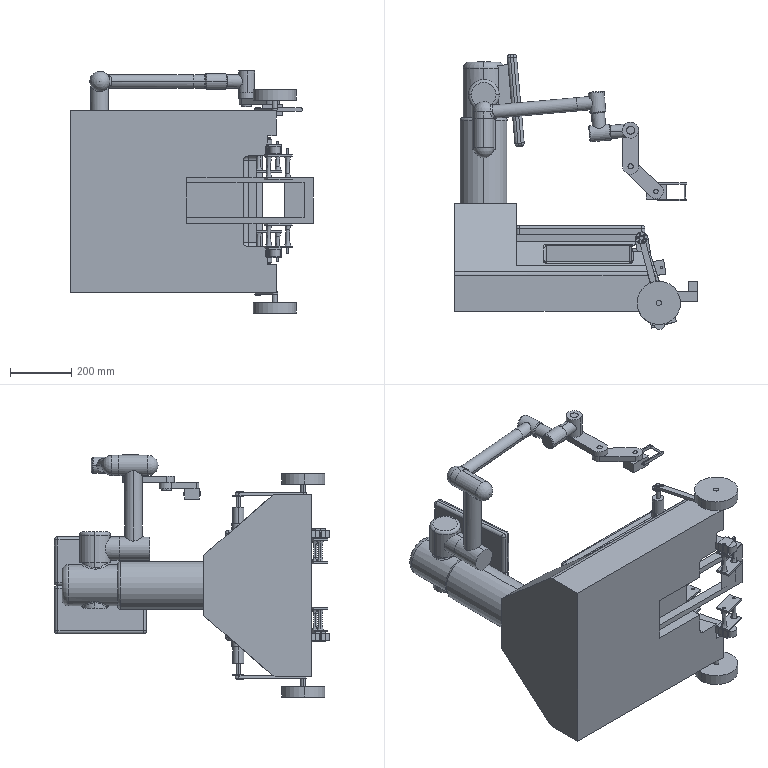Assembly | SolidWorks | mm | 23 component files | 62 solids | 754 faces | box 790.36 x 897.02 x 789.16 mm | volume 104777341 mm3 | plane 350 | cylinder 330 | spline 32 | sphere 28 | cone 8 | torus 6 | commonest cylinder face diameters 7.212 x34 20 x32 5.358 x32 8.088 x32 10 x18 12.936 x16 52.026 x9 43.427 x8
Bill of materials:
Joint | 1 |  | Multi-body articulated arrangement: a large flat circular disc on a short vertical post, a long thin flat link to a small perforated flange plate, a vertical cylinder housing, and a chain of flat rounded-end arm bars. Two plate pairs with waisted posts between them sit under the arm.
MirrorJoint | 1 |  | Multi-body articulated arrangement that appears geometrically the same as unnamed part but is shown inverted: large circular disc, post, long flat link, perforated flange, cylinder housing, rounded-end arm bars, and plate pairs with waisted posts.
RehabilitationChair-18-10 | 1 |  | Tee-like tubular junction: a thick-walled hollow cylinder with a solid cylindrical branch joining its side at an angle.
RehabilitationChair-18-1 | 1 |  | Thin flat rectangular plate with small rounded corners and slightly rounded edges.
RehabilitationChair-18-11 | 1 |  | Flanged cylindrical pin: a solid cylindrical shank standing on a larger, thin circular flange.
RehabilitationChair-18-13 | 1 |  | Plain solid cylindrical rod with flat ends.
RehabilitationChair-18-14 | 2 |  | Long thin flat bar with fully rounded ends and a single small through-hole near one end.
RehabilitationChair-18-15 | 1 |  | Complex blocky body: a large rectangular slab with stepped and chamfered edges, a protruding cylindrical boss on top, a recessed rounded-rectangle pocket, and a small pin-like feature along one edge.
RehabilitationChair-18-16 | 1 |  | Flat obround link plate with two equal small through-holes, one near each rounded end.
RehabilitationChair-18-17 | 1 |  | Solid rectangular block with one round through-hole off-centre on its largest face.
RehabilitationChair-18-18 | 1 |  | Thick obround link plate with two through-holes of different sizes, one near each rounded end.
RehabilitationChair-18-19 | 1 |  | Cylindrical rod whose end merges into a square block, with a short cylindrical cross-boss running perpendicular through the block region.
RehabilitationChair-18-2 | 1 |  | Two identical thin rectangular plates with rounded edges, placed edge to edge in one plane so together they form a larger rectangular panel.
RehabilitationChair-18-3 | 1 |  | Solid vertical cylinder with a rounded top edge, plus a smaller solid cylindrical boss sticking out sideways at right angles, ending in a flat face.
RehabilitationChair-18-4 | 1 |  | Solid hemisphere (half-sphere) with one flat circular face.
RehabilitationChair-18-5 | 2 |  | Tee-shaped solid made of a main cylinder with chamfered ends and a smaller cylindrical branch joined at right angles to its side.
RehabilitationChair-18-6 | 1 |  | Long, slender cylindrical rod with a larger rounded head at one end; the head has one flat face. A fillet blends the head into the shaft.
RehabilitationChair-18-7 | 1 |  | Plain solid cylindrical rod with flat ends.
RehabilitationChair-18-8 | 1 |  | Dumbbell or I-shaped solid: two short parallel cylinders joined by a perpendicular cylindrical bar.
RehabilitationChair-18-9 | 1 |  | Cylindrical pin with a thin, larger-diameter flange or collar at one end.
w | 1 |  | Fork- or U-shaped part with sharp edges and rectangular cross-sections: two parallel flat prongs joined at one end by a taller rectangular block, open at the other end.
Mates:
1. concentric | RehabilitationChair-18-15-1 face at (358.991, 36.933, 233) dir (0, 0, -1) r 10.044 | Joint-1 face at (358.991, 36.933, 180) dir (0, 0, 1) r 20.727
2. coincident | RehabilitationChair-18-15-1 face at (-203.591, 0, 180) dir (0, 0, 1) | Joint-1 face at (358.991, 36.933, 180) dir (0, 0, -1)